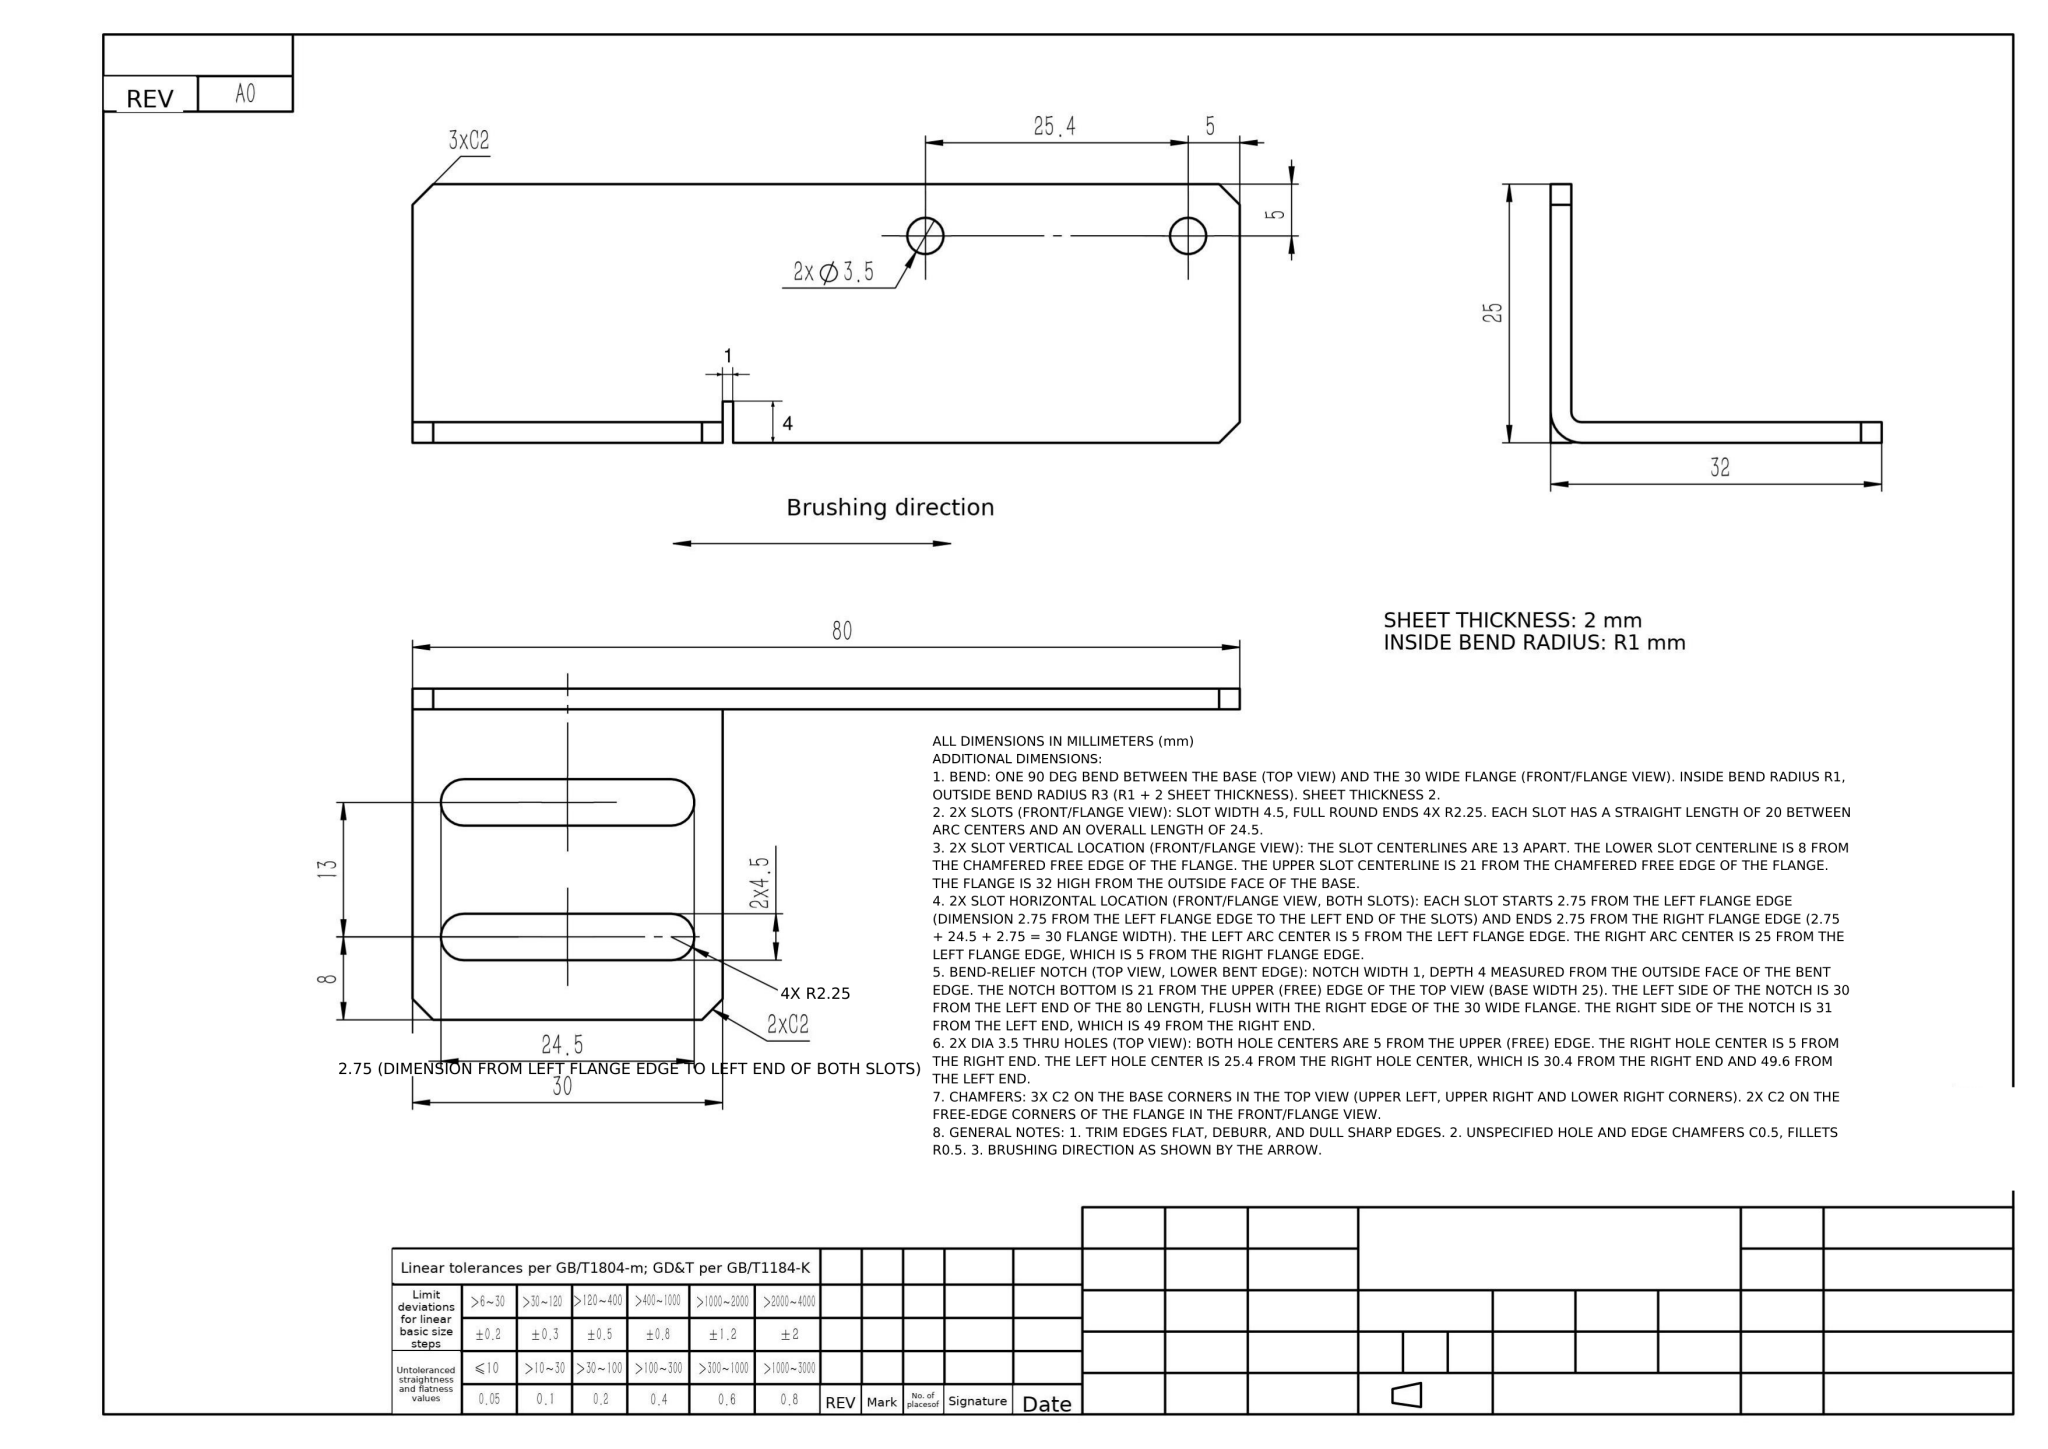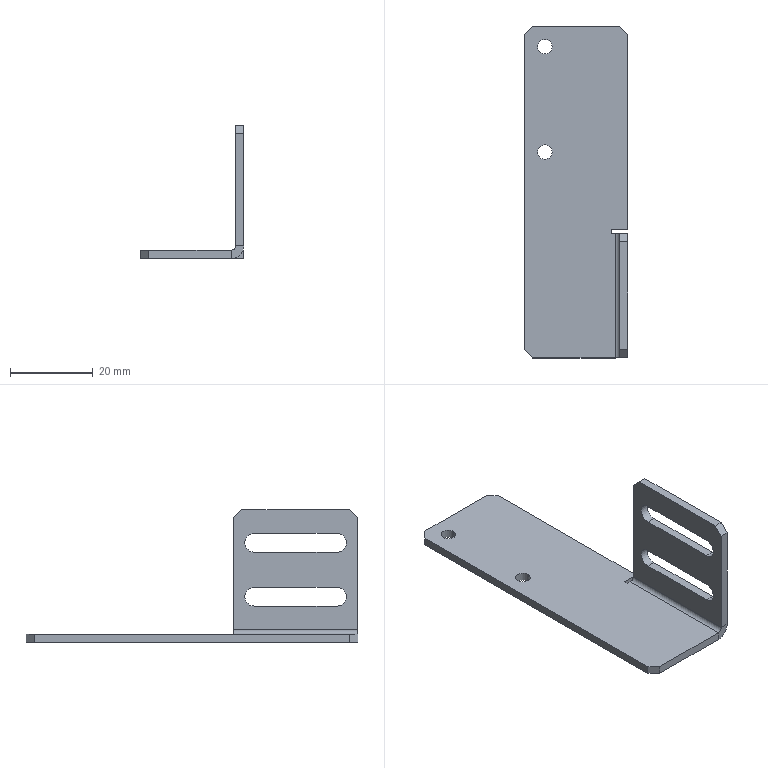Part | NX | mm | 1 solid | 35 faces | box 25 x 80 x 32 mm | volume 5258 mm3 | plane 25 | cylinder 10 | commonest cylinder face diameters 3.5 x4 4.5 x4 6 x1 2 x1